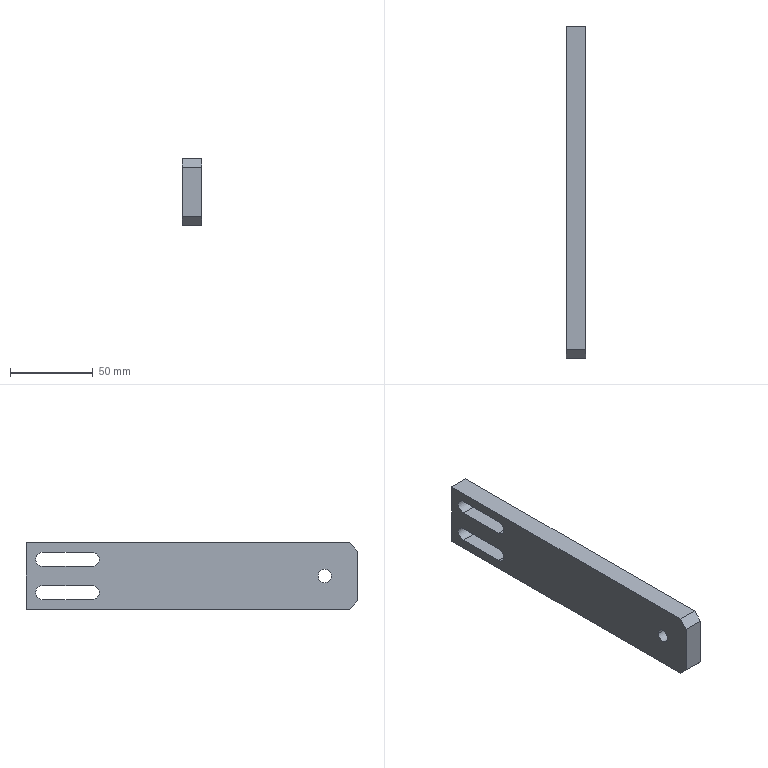Component | SolidWorks | ElectricalBoxAssembly2-1_GuidePlate2-1 | 1 solid | 20 faces | box 12 x 200 x 40 mm | volume 87615 mm3 | plane 12 | cylinder 8 | commonest cylinder face diameters 8.5 x6 8 x2
build123d program:
from build123d import *

# Parameters (mm, degrees)
SKETCH1_W           = 200
SKETCH1_H           = 40
BOSS_EXTRUDE1_DEPTH = 12
M8_TAPPED_HOLE1_D   = 8
CHAMFER1_SIZE       = 5
CHAMFER2_SIZE       = 5


with BuildPart() as part:
    # Sketch1 → Boss-Extrude1 (new body)
    with BuildSketch(Plane.XY):
        Rectangle(SKETCH1_W, SKETCH1_H)
        with BuildLine():
            Line((60, 14.25), (90, 14.25))
            ThreePointArc((90, 14.25), (94.25, 10), (90, 5.75))
            Line((90, 5.75), (60, 5.75))
            ThreePointArc((60, 5.75), (55.75, 10), (60, 14.25))
        make_face(mode=Mode.SUBTRACT)
        with BuildLine():
            Line((60, -5.75), (90, -5.75))
            ThreePointArc((90, -5.75), (94.25, -10), (90, -14.25))
            Line((90, -14.25), (60, -14.25))
            ThreePointArc((60, -14.25), (55.75, -10), (60, -5.75))
        make_face(mode=Mode.SUBTRACT)
    extrude(amount=BOSS_EXTRUDE1_DEPTH)

    # M8 Tapped Hole1 (through all)
    with Locations(Plane.XY.offset(12)):
        with Locations((-80, 0)):
            Hole(M8_TAPPED_HOLE1_D / 2)

    # Chamfer1
    chamfer1_edges = [part.edges().sort_by_distance(p)[0] for p in [
        (-100, 20, 6),
    ]]
    chamfer(chamfer1_edges, length=CHAMFER1_SIZE)

    # Chamfer2
    chamfer2_edges = [part.edges().sort_by_distance(p)[0] for p in [
        (-100, -20, 6),
    ]]
    chamfer(chamfer2_edges, length=CHAMFER2_SIZE)


solid = part.part

# Placed as in the assembly
solid = solid.moved(Location((743.468, 14.666, 1576.399), (90, 90, 0)))
STEP:
#1=CARTESIAN_POINT('',(29.743,-2.73,62.063));
#2=VERTEX_POINT('',#1);
#3=CARTESIAN_POINT('',(29.743,-2.415,62.063));
#4=VERTEX_POINT('',#3);
#5=CARTESIAN_POINT('',(29.743,-2.572,62.063));
#6=DIRECTION('',(-1.,-0.,-0.));
#7=DIRECTION('',(0.,1.,0.));
#8=AXIS2_PLACEMENT_3D('',#5,#6,#7);
#9=CIRCLE('',#8,0.1575);
#10=EDGE_CURVE('',#2,#4,#9,.T.);
#11=ORIENTED_EDGE('',*,*,#10,.F.);
#12=CARTESIAN_POINT('',(29.27,-2.73,62.063));
#13=VERTEX_POINT('',#12);
#14=CARTESIAN_POINT('',(29.27,-2.73,62.063));
#15=DIRECTION('',(-1.,-0.,-0.));
#16=VECTOR('',#15,39.37);
#17=LINE('',#14,#16);
#18=EDGE_CURVE('',#2,#13,#17,.T.);
#19=ORIENTED_EDGE('',*,*,#18,.T.);
#20=CARTESIAN_POINT('',(29.27,-2.415,62.063));
#21=VERTEX_POINT('',#20);
#22=CARTESIAN_POINT('',(29.27,-2.572,62.063));
#23=DIRECTION('',(-1.,-0.,-0.));
#24=DIRECTION('',(0.,1.,0.));
#25=AXIS2_PLACEMENT_3D('',#22,#23,#24);
#26=CIRCLE('',#25,0.1575);
#27=EDGE_CURVE('',#13,#21,#26,.T.);
#28=ORIENTED_EDGE('',*,*,#27,.T.);
#29=CARTESIAN_POINT('',(29.27,-2.415,62.063));
#30=DIRECTION('',(-1.,-0.,-0.));
#31=VECTOR('',#30,39.37);
#32=LINE('',#29,#31);
#33=EDGE_CURVE('',#4,#21,#32,.T.);
#34=ORIENTED_EDGE('',*,*,#33,.F.);
#35=EDGE_LOOP('',(#11,#19,#28,#34));
#36=FACE_OUTER_BOUND('',#35,.T.);
#37=CARTESIAN_POINT('',(29.27,-2.572,62.063));
#38=DIRECTION('',(-1.,-0.,-0.));
#39=DIRECTION('',(0.,1.,0.));
#40=AXIS2_PLACEMENT_3D('',#37,#38,#39);
#41=CYLINDRICAL_SURFACE('',#40,0.1575);
#42=ADVANCED_FACE('',(#36),#41,.F.);
#43=CARTESIAN_POINT('',(29.27,2.94,62.289));
#44=VERTEX_POINT('',#43);
#45=CARTESIAN_POINT('',(29.27,2.772,62.457));
#46=VERTEX_POINT('',#45);
#47=CARTESIAN_POINT('',(29.27,2.94,62.457));
#48=DIRECTION('',(-1.,-0.,-0.));
#49=DIRECTION('',(0.,1.,0.));
#50=AXIS2_PLACEMENT_3D('',#47,#48,#49);
#51=CIRCLE('',#50,0.1673);
#52=EDGE_CURVE('',#44,#46,#51,.T.);
#53=ORIENTED_EDGE('',*,*,#52,.T.);
#54=CARTESIAN_POINT('',(29.743,2.772,62.457));
#55=VERTEX_POINT('',#54);
#56=CARTESIAN_POINT('',(29.27,2.772,62.457));
#57=DIRECTION('',(1.,0.,0.));
#58=VECTOR('',#57,39.37);
#59=LINE('',#56,#58);
#60=EDGE_CURVE('',#46,#55,#59,.T.);
#61=ORIENTED_EDGE('',*,*,#60,.T.);
#62=CARTESIAN_POINT('',(29.743,2.94,62.289));
#63=VERTEX_POINT('',#62);
#64=CARTESIAN_POINT('',(29.743,2.94,62.457));
#65=DIRECTION('',(-1.,-0.,-0.));
#66=DIRECTION('',(0.,1.,0.));
#67=AXIS2_PLACEMENT_3D('',#64,#65,#66);
#68=CIRCLE('',#67,0.1673);
#69=EDGE_CURVE('',#63,#55,#68,.T.);
#70=ORIENTED_EDGE('',*,*,#69,.F.);
#71=CARTESIAN_POINT('',(29.27,2.94,62.289));
#72=DIRECTION('',(1.,0.,0.));
#73=VECTOR('',#72,39.37);
#74=LINE('',#71,#73);
#75=EDGE_CURVE('',#44,#63,#74,.T.);
#76=ORIENTED_EDGE('',*,*,#75,.F.);
#77=EDGE_LOOP('',(#53,#61,#70,#76));
#78=FACE_OUTER_BOUND('',#77,.T.);
#79=CARTESIAN_POINT('',(29.27,2.94,62.457));
#80=DIRECTION('',(1.,0.,0.));
#81=DIRECTION('',(0.,-1.,0.));
#82=AXIS2_PLACEMENT_3D('',#79,#80,#81);
#83=CYLINDRICAL_SURFACE('',#82,0.1673);
#84=ADVANCED_FACE('',(#78),#83,.F.);
#85=CARTESIAN_POINT('',(29.27,2.94,61.502));
#86=VERTEX_POINT('',#85);
#87=CARTESIAN_POINT('',(29.27,2.772,61.669));
#88=VERTEX_POINT('',#87);
#89=CARTESIAN_POINT('',(29.27,2.94,61.669));
#90=DIRECTION('',(-1.,-0.,-0.));
#91=DIRECTION('',(0.,1.,0.));
#92=AXIS2_PLACEMENT_3D('',#89,#90,#91);
#93=CIRCLE('',#92,0.1673);
#94=EDGE_CURVE('',#86,#88,#93,.T.);
#95=ORIENTED_EDGE('',*,*,#94,.T.);
#96=CARTESIAN_POINT('',(29.743,2.772,61.669));
#97=VERTEX_POINT('',#96);
#98=CARTESIAN_POINT('',(29.27,2.772,61.669));
#99=DIRECTION('',(1.,0.,0.));
#100=VECTOR('',#99,39.37);
#101=LINE('',#98,#100);
#102=EDGE_CURVE('',#88,#97,#101,.T.);
#103=ORIENTED_EDGE('',*,*,#102,.T.);
#104=CARTESIAN_POINT('',(29.743,2.94,61.502));
#105=VERTEX_POINT('',#104);
#106=CARTESIAN_POINT('',(29.743,2.94,61.669));
#107=DIRECTION('',(-1.,-0.,-0.));
#108=DIRECTION('',(0.,1.,0.));
#109=AXIS2_PLACEMENT_3D('',#106,#107,#108);
#110=CIRCLE('',#109,0.1673);
#111=EDGE_CURVE('',#105,#97,#110,.T.);
#112=ORIENTED_EDGE('',*,*,#111,.F.);
#113=CARTESIAN_POINT('',(29.27,2.94,61.502));
#114=DIRECTION('',(1.,0.,0.));
#115=VECTOR('',#114,39.37);
#116=LINE('',#113,#115);
#117=EDGE_CURVE('',#86,#105,#116,.T.);
#118=ORIENTED_EDGE('',*,*,#117,.F.);
#119=EDGE_LOOP('',(#95,#103,#112,#118));
#120=FACE_OUTER_BOUND('',#119,.T.);
#121=CARTESIAN_POINT('',(29.27,2.94,61.669));
#122=DIRECTION('',(1.,0.,0.));
#123=DIRECTION('',(0.,-1.,0.));
#124=AXIS2_PLACEMENT_3D('',#121,#122,#123);
#125=CYLINDRICAL_SURFACE('',#124,0.1673);
#126=ADVANCED_FACE('',(#120),#125,.F.);
#127=CARTESIAN_POINT('',(29.27,-2.572,62.063));
#128=DIRECTION('',(-1.,-0.,-0.));
#129=DIRECTION('',(0.,1.,0.));
#130=AXIS2_PLACEMENT_3D('',#127,#128,#129);
#131=CIRCLE('',#130,0.1575);
#132=EDGE_CURVE('',#21,#13,#131,.T.);
#133=ORIENTED_EDGE('',*,*,#132,.F.);
#134=ORIENTED_EDGE('',*,*,#27,.F.);
#135=EDGE_LOOP('',(#133,#134));
#136=FACE_BOUND('',#135,.T.);
#137=CARTESIAN_POINT('',(29.27,-3.36,61.472));
#138=VERTEX_POINT('',#137);
#139=CARTESIAN_POINT('',(29.27,-3.36,62.653));
#140=VERTEX_POINT('',#139);
#141=CARTESIAN_POINT('',(29.27,-3.36,61.276));
#142=DIRECTION('',(-0.,-0.,1.));
#143=VECTOR('',#142,39.37);
#144=LINE('',#141,#143);
#145=EDGE_CURVE('',#138,#140,#144,.T.);
#146=ORIENTED_EDGE('',*,*,#145,.T.);
#147=CARTESIAN_POINT('',(29.27,-3.163,62.85));
#148=VERTEX_POINT('',#147);
#149=CARTESIAN_POINT('',(29.27,-1.686,64.327));
#150=DIRECTION('',(-0.,0.7071,0.7071));
#151=VECTOR('',#150,39.37);
#152=LINE('',#149,#151);
#153=EDGE_CURVE('',#140,#148,#152,.T.);
#154=ORIENTED_EDGE('',*,*,#153,.T.);
#155=CARTESIAN_POINT('',(29.27,4.514,62.85));
#156=VERTEX_POINT('',#155);
#157=CARTESIAN_POINT('',(29.27,-3.36,62.85));
#158=DIRECTION('',(-0.,1.,0.));
#159=VECTOR('',#158,39.37);
#160=LINE('',#157,#159);
#161=EDGE_CURVE('',#148,#156,#160,.T.);
#162=ORIENTED_EDGE('',*,*,#161,.T.);
#163=CARTESIAN_POINT('',(29.27,4.514,61.276));
#164=VERTEX_POINT('',#163);
#165=CARTESIAN_POINT('',(29.27,4.514,61.276));
#166=DIRECTION('',(0.,0.,-1.));
#167=VECTOR('',#166,39.37);
#168=LINE('',#165,#167);
#169=EDGE_CURVE('',#156,#164,#168,.T.);
#170=ORIENTED_EDGE('',*,*,#169,.T.);
#171=CARTESIAN_POINT('',(29.27,-3.163,61.276));
#172=VERTEX_POINT('',#171);
#173=CARTESIAN_POINT('',(29.27,-3.36,61.276));
#174=DIRECTION('',(0.,-1.,-0.));
#175=VECTOR('',#174,39.37);
#176=LINE('',#173,#175);
#177=EDGE_CURVE('',#164,#172,#176,.T.);
#178=ORIENTED_EDGE('',*,*,#177,.T.);
#179=CARTESIAN_POINT('',(29.27,-1.686,59.799));
#180=DIRECTION('',(-0.,-0.7071,0.7071));
#181=VECTOR('',#180,39.37);
#182=LINE('',#179,#181);
#183=EDGE_CURVE('',#172,#138,#182,.T.);
#184=ORIENTED_EDGE('',*,*,#183,.T.);
#185=EDGE_LOOP('',(#146,#154,#162,#170,#178,#184));
#186=FACE_OUTER_BOUND('',#185,.T.);
#187=CARTESIAN_POINT('',(29.27,2.94,61.837));
#188=VERTEX_POINT('',#187);
#189=CARTESIAN_POINT('',(29.27,4.121,61.837));
#190=VERTEX_POINT('',#189);
#191=CARTESIAN_POINT('',(29.27,2.94,61.837));
#192=DIRECTION('',(-0.,1.,0.));
#193=VECTOR('',#192,39.37);
#194=LINE('',#191,#193);
#195=EDGE_CURVE('',#188,#190,#194,.T.);
#196=ORIENTED_EDGE('',*,*,#195,.F.);
#197=CARTESIAN_POINT('',(29.27,2.94,61.669));
#198=DIRECTION('',(-1.,-0.,-0.));
#199=DIRECTION('',(0.,1.,0.));
#200=AXIS2_PLACEMENT_3D('',#197,#198,#199);
#201=CIRCLE('',#200,0.1673);
#202=EDGE_CURVE('',#88,#188,#201,.T.);
#203=ORIENTED_EDGE('',*,*,#202,.F.);
#204=ORIENTED_EDGE('',*,*,#94,.F.);
#205=CARTESIAN_POINT('',(29.27,4.121,61.502));
#206=VERTEX_POINT('',#205);
#207=CARTESIAN_POINT('',(29.27,2.94,61.502));
#208=DIRECTION('',(0.,-1.,-0.));
#209=VECTOR('',#208,39.37);
#210=LINE('',#207,#209);
#211=EDGE_CURVE('',#206,#86,#210,.T.);
#212=ORIENTED_EDGE('',*,*,#211,.F.);
#213=CARTESIAN_POINT('',(29.27,4.121,61.669));
#214=DIRECTION('',(-1.,-0.,-0.));
#215=DIRECTION('',(0.,1.,0.));
#216=AXIS2_PLACEMENT_3D('',#213,#214,#215);
#217=CIRCLE('',#216,0.1673);
#218=EDGE_CURVE('',#190,#206,#217,.T.);
#219=ORIENTED_EDGE('',*,*,#218,.F.);
#220=EDGE_LOOP('',(#196,#203,#204,#212,#219));
#221=FACE_BOUND('',#220,.T.);
#222=CARTESIAN_POINT('',(29.27,2.94,62.624));
#223=VERTEX_POINT('',#222);
#224=CARTESIAN_POINT('',(29.27,4.121,62.624));
#225=VERTEX_POINT('',#224);
#226=CARTESIAN_POINT('',(29.27,2.94,62.624));
#227=DIRECTION('',(-0.,1.,0.));
#228=VECTOR('',#227,39.37);
#229=LINE('',#226,#228);
#230=EDGE_CURVE('',#223,#225,#229,.T.);
#231=ORIENTED_EDGE('',*,*,#230,.F.);
#232=CARTESIAN_POINT('',(29.27,2.94,62.457));
#233=DIRECTION('',(-1.,-0.,-0.));
#234=DIRECTION('',(0.,1.,0.));
#235=AXIS2_PLACEMENT_3D('',#232,#233,#234);
#236=CIRCLE('',#235,0.1673);
#237=EDGE_CURVE('',#46,#223,#236,.T.);
#238=ORIENTED_EDGE('',*,*,#237,.F.);
#239=ORIENTED_EDGE('',*,*,#52,.F.);
#240=CARTESIAN_POINT('',(29.27,4.121,62.289));
#241=VERTEX_POINT('',#240);
#242=CARTESIAN_POINT('',(29.27,2.94,62.289));
#243=DIRECTION('',(0.,-1.,-0.));
#244=VECTOR('',#243,39.37);
#245=LINE('',#242,#244);
#246=EDGE_CURVE('',#241,#44,#245,.T.);
#247=ORIENTED_EDGE('',*,*,#246,.F.);
#248=CARTESIAN_POINT('',(29.27,4.121,62.457));
#249=DIRECTION('',(-1.,-0.,-0.));
#250=DIRECTION('',(0.,1.,0.));
#251=AXIS2_PLACEMENT_3D('',#248,#249,#250);
#252=CIRCLE('',#251,0.1673);
#253=EDGE_CURVE('',#225,#241,#252,.T.);
#254=ORIENTED_EDGE('',*,*,#253,.F.);
#255=EDGE_LOOP('',(#231,#238,#239,#247,#254));
#256=FACE_BOUND('',#255,.T.);
#257=CARTESIAN_POINT('',(29.27,0.5774,62.063));
#258=DIRECTION('',(-1.,-0.,-0.));
#259=DIRECTION('',(-0.,1.,0.));
#260=AXIS2_PLACEMENT_3D('',#257,#258,#259);
#261=PLANE('',#260);
#262=ADVANCED_FACE('',(#136,#186,#221,#256),#261,.T.);
#263=CARTESIAN_POINT('',(29.743,-2.572,62.063));
#264=DIRECTION('',(-1.,-0.,-0.));
#265=DIRECTION('',(0.,1.,0.));
#266=AXIS2_PLACEMENT_3D('',#263,#264,#265);
#267=CIRCLE('',#266,0.1575);
#268=EDGE_CURVE('',#4,#2,#267,.T.);
#269=ORIENTED_EDGE('',*,*,#268,.T.);
#270=ORIENTED_EDGE('',*,*,#10,.T.);
#271=EDGE_LOOP('',(#269,#270));
#272=FACE_BOUND('',#271,.T.);
#273=ORIENTED_EDGE('',*,*,#111,.T.);
#274=CARTESIAN_POINT('',(29.743,2.94,61.837));
#275=VERTEX_POINT('',#274);
#276=CARTESIAN_POINT('',(29.743,2.94,61.669));
#277=DIRECTION('',(-1.,-0.,-0.));
#278=DIRECTION('',(0.,1.,0.));
#279=AXIS2_PLACEMENT_3D('',#276,#277,#278);
#280=CIRCLE('',#279,0.1673);
#281=EDGE_CURVE('',#97,#275,#280,.T.);
#282=ORIENTED_EDGE('',*,*,#281,.T.);
#283=CARTESIAN_POINT('',(29.743,4.121,61.837));
#284=VERTEX_POINT('',#283);
#285=CARTESIAN_POINT('',(29.743,2.94,61.837));
#286=DIRECTION('',(-0.,1.,0.));
#287=VECTOR('',#286,39.37);
#288=LINE('',#285,#287);
#289=EDGE_CURVE('',#275,#284,#288,.T.);
#290=ORIENTED_EDGE('',*,*,#289,.T.);
#291=CARTESIAN_POINT('',(29.743,4.121,61.502));
#292=VERTEX_POINT('',#291);
#293=CARTESIAN_POINT('',(29.743,4.121,61.669));
#294=DIRECTION('',(-1.,-0.,-0.));
#295=DIRECTION('',(0.,1.,0.));
#296=AXIS2_PLACEMENT_3D('',#293,#294,#295);
#297=CIRCLE('',#296,0.1673);
#298=EDGE_CURVE('',#284,#292,#297,.T.);
#299=ORIENTED_EDGE('',*,*,#298,.T.);
#300=CARTESIAN_POINT('',(29.743,2.94,61.502));
#301=DIRECTION('',(0.,-1.,-0.));
#302=VECTOR('',#301,39.37);
#303=LINE('',#300,#302);
#304=EDGE_CURVE('',#292,#105,#303,.T.);
#305=ORIENTED_EDGE('',*,*,#304,.T.);
#306=EDGE_LOOP('',(#273,#282,#290,#299,#305));
#307=FACE_BOUND('',#306,.T.);
#308=CARTESIAN_POINT('',(29.743,-3.163,62.85));
#309=VERTEX_POINT('',#308);
#310=CARTESIAN_POINT('',(29.743,4.514,62.85));
#311=VERTEX_POINT('',#310);
#312=CARTESIAN_POINT('',(29.743,-3.36,62.85));
#313=DIRECTION('',(-0.,1.,0.));
#314=VECTOR('',#313,39.37);
#315=LINE('',#312,#314);
#316=EDGE_CURVE('',#309,#311,#315,.T.);
#317=ORIENTED_EDGE('',*,*,#316,.F.);
#318=CARTESIAN_POINT('',(29.743,-3.36,62.653));
#319=VERTEX_POINT('',#318);
#320=CARTESIAN_POINT('',(29.743,-3.163,62.85));
#321=DIRECTION('',(0.,-0.7071,-0.7071));
#322=VECTOR('',#321,39.37);
#323=LINE('',#320,#322);
#324=EDGE_CURVE('',#309,#319,#323,.T.);
#325=ORIENTED_EDGE('',*,*,#324,.T.);
#326=CARTESIAN_POINT('',(29.743,-3.36,61.472));
#327=VERTEX_POINT('',#326);
#328=CARTESIAN_POINT('',(29.743,-3.36,61.276));
#329=DIRECTION('',(-0.,-0.,1.));
#330=VECTOR('',#329,39.37);
#331=LINE('',#328,#330);
#332=EDGE_CURVE('',#327,#319,#331,.T.);
#333=ORIENTED_EDGE('',*,*,#332,.F.);
#334=CARTESIAN_POINT('',(29.743,-3.163,61.276));
#335=VERTEX_POINT('',#334);
#336=CARTESIAN_POINT('',(29.743,-3.36,61.472));
#337=DIRECTION('',(0.,0.7071,-0.7071));
#338=VECTOR('',#337,39.37);
#339=LINE('',#336,#338);
#340=EDGE_CURVE('',#327,#335,#339,.T.);
#341=ORIENTED_EDGE('',*,*,#340,.T.);
#342=CARTESIAN_POINT('',(29.743,4.514,61.276));
#343=VERTEX_POINT('',#342);
#344=CARTESIAN_POINT('',(29.743,-3.36,61.276));
#345=DIRECTION('',(0.,-1.,-0.));
#346=VECTOR('',#345,39.37);
#347=LINE('',#344,#346);
#348=EDGE_CURVE('',#343,#335,#347,.T.);
#349=ORIENTED_EDGE('',*,*,#348,.F.);
#350=CARTESIAN_POINT('',(29.743,4.514,61.276));
#351=DIRECTION('',(0.,0.,-1.));
#352=VECTOR('',#351,39.37);
#353=LINE('',#350,#352);
#354=EDGE_CURVE('',#311,#343,#353,.T.);
#355=ORIENTED_EDGE('',*,*,#354,.F.);
#356=EDGE_LOOP('',(#317,#325,#333,#341,#349,#355));
#357=FACE_OUTER_BOUND('',#356,.T.);
#358=ORIENTED_EDGE('',*,*,#69,.T.);
#359=CARTESIAN_POINT('',(29.743,2.94,62.624));
#360=VERTEX_POINT('',#359);
#361=CARTESIAN_POINT('',(29.743,2.94,62.457));
#362=DIRECTION('',(-1.,-0.,-0.));
#363=DIRECTION('',(0.,1.,0.));
#364=AXIS2_PLACEMENT_3D('',#361,#362,#363);
#365=CIRCLE('',#364,0.1673);
#366=EDGE_CURVE('',#55,#360,#365,.T.);
#367=ORIENTED_EDGE('',*,*,#366,.T.);
#368=CARTESIAN_POINT('',(29.743,4.121,62.624));
#369=VERTEX_POINT('',#368);
#370=CARTESIAN_POINT('',(29.743,2.94,62.624));
#371=DIRECTION('',(-0.,1.,0.));
#372=VECTOR('',#371,39.37);
#373=LINE('',#370,#372);
#374=EDGE_CURVE('',#360,#369,#373,.T.);
#375=ORIENTED_EDGE('',*,*,#374,.T.);
#376=CARTESIAN_POINT('',(29.743,4.121,62.289));
#377=VERTEX_POINT('',#376);
#378=CARTESIAN_POINT('',(29.743,4.121,62.457));
#379=DIRECTION('',(-1.,-0.,-0.));
#380=DIRECTION('',(0.,1.,0.));
#381=AXIS2_PLACEMENT_3D('',#378,#379,#380);
#382=CIRCLE('',#381,0.1673);
#383=EDGE_CURVE('',#369,#377,#382,.T.);
#384=ORIENTED_EDGE('',*,*,#383,.T.);
#385=CARTESIAN_POINT('',(29.743,2.94,62.289));
#386=DIRECTION('',(0.,-1.,-0.));
#387=VECTOR('',#386,39.37);
#388=LINE('',#385,#387);
#389=EDGE_CURVE('',#377,#63,#388,.T.);
#390=ORIENTED_EDGE('',*,*,#389,.T.);
#391=EDGE_LOOP('',(#358,#367,#375,#384,#390));
#392=FACE_BOUND('',#391,.T.);
#393=CARTESIAN_POINT('',(29.743,0.5774,62.063));
#394=DIRECTION('',(-1.,-0.,-0.));
#395=DIRECTION('',(-0.,1.,0.));
#396=AXIS2_PLACEMENT_3D('',#393,#394,#395);
#397=PLANE('',#396);
#398=ADVANCED_FACE('',(#272,#307,#357,#392),#397,.F.);
#399=ORIENTED_EDGE('',*,*,#354,.T.);
#400=CARTESIAN_POINT('',(29.27,4.514,61.276));
#401=DIRECTION('',(1.,0.,0.));
#402=VECTOR('',#401,39.37);
#403=LINE('',#400,#402);
#404=EDGE_CURVE('',#164,#343,#403,.T.);
#405=ORIENTED_EDGE('',*,*,#404,.F.);
#406=ORIENTED_EDGE('',*,*,#169,.F.);
#407=CARTESIAN_POINT('',(29.27,4.514,62.85));
#408=DIRECTION('',(1.,0.,0.));
#409=VECTOR('',#408,39.37);
#410=LINE('',#407,#409);
#411=EDGE_CURVE('',#156,#311,#410,.T.);
#412=ORIENTED_EDGE('',*,*,#411,.T.);
#413=EDGE_LOOP('',(#399,#405,#406,#412));
#414=FACE_OUTER_BOUND('',#413,.T.);
#415=CARTESIAN_POINT('',(29.27,4.514,61.276));
#416=DIRECTION('',(0.,-1.,-0.));
#417=DIRECTION('',(-1.,-0.,-0.));
#418=AXIS2_PLACEMENT_3D('',#415,#416,#417);
#419=PLANE('',#418);
#420=ADVANCED_FACE('',(#414),#419,.F.);
#421=ORIENTED_EDGE('',*,*,#348,.T.);
#422=CARTESIAN_POINT('',(29.27,-3.163,61.276));
#423=DIRECTION('',(-1.,-0.,-0.));
#424=VECTOR('',#423,39.37);
#425=LINE('',#422,#424);
#426=EDGE_CURVE('',#335,#172,#425,.T.);
#427=ORIENTED_EDGE('',*,*,#426,.T.);
#428=ORIENTED_EDGE('',*,*,#177,.F.);
#429=ORIENTED_EDGE('',*,*,#404,.T.);
#430=EDGE_LOOP('',(#421,#427,#428,#429));
#431=FACE_OUTER_BOUND('',#430,.T.);
#432=CARTESIAN_POINT('',(29.27,-3.36,61.276));
#433=DIRECTION('',(-0.,-0.,1.));
#434=DIRECTION('',(1.,0.,0.));
#435=AXIS2_PLACEMENT_3D('',#432,#433,#434);
#436=PLANE('',#435);
#437=ADVANCED_FACE('',(#431),#436,.F.);
#438=ORIENTED_EDGE('',*,*,#332,.T.);
#439=CARTESIAN_POINT('',(29.27,-3.36,62.653));
#440=DIRECTION('',(-1.,-0.,-0.));
#441=VECTOR('',#440,39.37);
#442=LINE('',#439,#441);
#443=EDGE_CURVE('',#319,#140,#442,.T.);
#444=ORIENTED_EDGE('',*,*,#443,.T.);
#445=ORIENTED_EDGE('',*,*,#145,.F.);
#446=CARTESIAN_POINT('',(29.27,-3.36,61.472));
#447=DIRECTION('',(1.,0.,0.));
#448=VECTOR('',#447,39.37);
#449=LINE('',#446,#448);
#450=EDGE_CURVE('',#138,#327,#449,.T.);
#451=ORIENTED_EDGE('',*,*,#450,.T.);
#452=EDGE_LOOP('',(#438,#444,#445,#451));
#453=FACE_OUTER_BOUND('',#452,.T.);
#454=CARTESIAN_POINT('',(29.27,-3.36,61.276));
#455=DIRECTION('',(-0.,1.,0.));
#456=DIRECTION('',(1.,0.,0.));
#457=AXIS2_PLACEMENT_3D('',#454,#455,#456);
#458=PLANE('',#457);
#459=ADVANCED_FACE('',(#453),#458,.F.);
#460=ORIENTED_EDGE('',*,*,#161,.F.);
#461=CARTESIAN_POINT('',(29.27,-3.163,62.85));
#462=DIRECTION('',(1.,0.,0.));
#463=VECTOR('',#462,39.37);
#464=LINE('',#461,#463);
#465=EDGE_CURVE('',#148,#309,#464,.T.);
#466=ORIENTED_EDGE('',*,*,#465,.T.);
#467=ORIENTED_EDGE('',*,*,#316,.T.);
#468=ORIENTED_EDGE('',*,*,#411,.F.);
#469=EDGE_LOOP('',(#460,#466,#467,#468));
#470=FACE_OUTER_BOUND('',#469,.T.);
#471=CARTESIAN_POINT('',(29.27,-3.36,62.85));
#472=DIRECTION('',(0.,0.,-1.));
#473=DIRECTION('',(-1.,-0.,-0.));
#474=AXIS2_PLACEMENT_3D('',#471,#472,#473);
#475=PLANE('',#474);
#476=ADVANCED_FACE('',(#470),#475,.F.);
#477=ORIENTED_EDGE('',*,*,#102,.F.);
#478=ORIENTED_EDGE('',*,*,#202,.T.);
#479=CARTESIAN_POINT('',(29.27,2.94,61.837));
#480=DIRECTION('',(1.,0.,0.));
#481=VECTOR('',#480,39.37);
#482=LINE('',#479,#481);
#483=EDGE_CURVE('',#188,#275,#482,.T.);
#484=ORIENTED_EDGE('',*,*,#483,.T.);
#485=ORIENTED_EDGE('',*,*,#281,.F.);
#486=EDGE_LOOP('',(#477,#478,#484,#485));
#487=FACE_OUTER_BOUND('',#486,.T.);
#488=CARTESIAN_POINT('',(29.27,2.94,61.669));
#489=DIRECTION('',(1.,0.,0.));
#490=DIRECTION('',(0.,-1.,0.));
#491=AXIS2_PLACEMENT_3D('',#488,#489,#490);
#492=CYLINDRICAL_SURFACE('',#491,0.1673);
#493=ADVANCED_FACE('',(#487),#492,.F.);
#494=ORIENTED_EDGE('',*,*,#289,.F.);
#495=ORIENTED_EDGE('',*,*,#483,.F.);
#496=ORIENTED_EDGE('',*,*,#195,.T.);
#497=CARTESIAN_POINT('',(29.27,4.121,61.837));
#498=DIRECTION('',(1.,0.,0.));
#499=VECTOR('',#498,39.37);
#500=LINE('',#497,#499);
#501=EDGE_CURVE('',#190,#284,#500,.T.);
#502=ORIENTED_EDGE('',*,*,#501,.T.);
#503=EDGE_LOOP('',(#494,#495,#496,#502));
#504=FACE_OUTER_BOUND('',#503,.T.);
#505=CARTESIAN_POINT('',(29.27,2.94,61.837));
#506=DIRECTION('',(0.,0.,-1.));
#507=DIRECTION('',(-1.,-0.,-0.));
#508=AXIS2_PLACEMENT_3D('',#505,#506,#507);
#509=PLANE('',#508);
#510=ADVANCED_FACE('',(#504),#509,.T.);
#511=ORIENTED_EDGE('',*,*,#298,.F.);
#512=ORIENTED_EDGE('',*,*,#501,.F.);
#513=ORIENTED_EDGE('',*,*,#218,.T.);
#514=CARTESIAN_POINT('',(29.27,4.121,61.502));
#515=DIRECTION('',(1.,0.,0.));
#516=VECTOR('',#515,39.37);
#517=LINE('',#514,#516);
#518=EDGE_CURVE('',#206,#292,#517,.T.);
#519=ORIENTED_EDGE('',*,*,#518,.T.);
#520=EDGE_LOOP('',(#511,#512,#513,#519));
#521=FACE_OUTER_BOUND('',#520,.T.);
#522=CARTESIAN_POINT('',(29.27,4.121,61.669));
#523=DIRECTION('',(1.,0.,0.));
#524=DIRECTION('',(0.,-1.,0.));
#525=AXIS2_PLACEMENT_3D('',#522,#523,#524);
#526=CYLINDRICAL_SURFACE('',#525,0.1673);
#527=ADVANCED_FACE('',(#521),#526,.F.);
#528=ORIENTED_EDGE('',*,*,#304,.F.);
#529=ORIENTED_EDGE('',*,*,#518,.F.);
#530=ORIENTED_EDGE('',*,*,#211,.T.);
#531=ORIENTED_EDGE('',*,*,#117,.T.);
#532=EDGE_LOOP('',(#528,#529,#530,#531));
#533=FACE_OUTER_BOUND('',#532,.T.);
#534=CARTESIAN_POINT('',(29.27,2.94,61.502));
#535=DIRECTION('',(-0.,-0.,1.));
#536=DIRECTION('',(1.,0.,0.));
#537=AXIS2_PLACEMENT_3D('',#534,#535,#536);
#538=PLANE('',#537);
#539=ADVANCED_FACE('',(#533),#538,.T.);
#540=ORIENTED_EDGE('',*,*,#60,.F.);
#541=ORIENTED_EDGE('',*,*,#237,.T.);
#542=CARTESIAN_POINT('',(29.27,2.94,62.624));
#543=DIRECTION('',(1.,0.,0.));
#544=VECTOR('',#543,39.37);
#545=LINE('',#542,#544);
#546=EDGE_CURVE('',#223,#360,#545,.T.);
#547=ORIENTED_EDGE('',*,*,#546,.T.);
#548=ORIENTED_EDGE('',*,*,#366,.F.);
#549=EDGE_LOOP('',(#540,#541,#547,#548));
#550=FACE_OUTER_BOUND('',#549,.T.);
#551=CARTESIAN_POINT('',(29.27,2.94,62.457));
#552=DIRECTION('',(1.,0.,0.));
#553=DIRECTION('',(0.,-1.,0.));
#554=AXIS2_PLACEMENT_3D('',#551,#552,#553);
#555=CYLINDRICAL_SURFACE('',#554,0.1673);
#556=ADVANCED_FACE('',(#550),#555,.F.);
#557=ORIENTED_EDGE('',*,*,#374,.F.);
#558=ORIENTED_EDGE('',*,*,#546,.F.);
#559=ORIENTED_EDGE('',*,*,#230,.T.);
#560=CARTESIAN_POINT('',(29.27,4.121,62.624));
#561=DIRECTION('',(1.,0.,0.));
#562=VECTOR('',#561,39.37);
#563=LINE('',#560,#562);
#564=EDGE_CURVE('',#225,#369,#563,.T.);
#565=ORIENTED_EDGE('',*,*,#564,.T.);
#566=EDGE_LOOP('',(#557,#558,#559,#565));
#567=FACE_OUTER_BOUND('',#566,.T.);
#568=CARTESIAN_POINT('',(29.27,2.94,62.624));
#569=DIRECTION('',(0.,0.,-1.));
#570=DIRECTION('',(-1.,-0.,-0.));
#571=AXIS2_PLACEMENT_3D('',#568,#569,#570);
#572=PLANE('',#571);
#573=ADVANCED_FACE('',(#567),#572,.T.);
#574=ORIENTED_EDGE('',*,*,#383,.F.);
#575=ORIENTED_EDGE('',*,*,#564,.F.);
#576=ORIENTED_EDGE('',*,*,#253,.T.);
#577=CARTESIAN_POINT('',(29.27,4.121,62.289));
#578=DIRECTION('',(1.,0.,0.));
#579=VECTOR('',#578,39.37);
#580=LINE('',#577,#579);
#581=EDGE_CURVE('',#241,#377,#580,.T.);
#582=ORIENTED_EDGE('',*,*,#581,.T.);
#583=EDGE_LOOP('',(#574,#575,#576,#582));
#584=FACE_OUTER_BOUND('',#583,.T.);
#585=CARTESIAN_POINT('',(29.27,4.121,62.457));
#586=DIRECTION('',(1.,0.,0.));
#587=DIRECTION('',(0.,-1.,0.));
#588=AXIS2_PLACEMENT_3D('',#585,#586,#587);
#589=CYLINDRICAL_SURFACE('',#588,0.1673);
#590=ADVANCED_FACE('',(#584),#589,.F.);
#591=ORIENTED_EDGE('',*,*,#389,.F.);
#592=ORIENTED_EDGE('',*,*,#581,.F.);
#593=ORIENTED_EDGE('',*,*,#246,.T.);
#594=ORIENTED_EDGE('',*,*,#75,.T.);
#595=EDGE_LOOP('',(#591,#592,#593,#594));
#596=FACE_OUTER_BOUND('',#595,.T.);
#597=CARTESIAN_POINT('',(29.27,2.94,62.289));
#598=DIRECTION('',(-0.,-0.,1.));
#599=DIRECTION('',(1.,0.,0.));
#600=AXIS2_PLACEMENT_3D('',#597,#598,#599);
#601=PLANE('',#600);
#602=ADVANCED_FACE('',(#596),#601,.T.);
#603=ORIENTED_EDGE('',*,*,#18,.F.);
#604=ORIENTED_EDGE('',*,*,#268,.F.);
#605=ORIENTED_EDGE('',*,*,#33,.T.);
#606=ORIENTED_EDGE('',*,*,#132,.T.);
#607=EDGE_LOOP('',(#603,#604,#605,#606));
#608=FACE_OUTER_BOUND('',#607,.T.);
#609=CARTESIAN_POINT('',(29.27,-2.572,62.063));
#610=DIRECTION('',(-1.,-0.,-0.));
#611=DIRECTION('',(0.,1.,0.));
#612=AXIS2_PLACEMENT_3D('',#609,#610,#611);
#613=CYLINDRICAL_SURFACE('',#612,0.1575);
#614=ADVANCED_FACE('',(#608),#613,.F.);
#615=ORIENTED_EDGE('',*,*,#183,.F.);
#616=ORIENTED_EDGE('',*,*,#426,.F.);
#617=ORIENTED_EDGE('',*,*,#340,.F.);
#618=ORIENTED_EDGE('',*,*,#450,.F.);
#619=EDGE_LOOP('',(#615,#616,#617,#618));
#620=FACE_OUTER_BOUND('',#619,.T.);
#621=CARTESIAN_POINT('',(29.27,-3.36,61.472));
#622=DIRECTION('',(-0.,0.7071,0.7071));
#623=DIRECTION('',(1.,0.,0.));
#624=AXIS2_PLACEMENT_3D('',#621,#622,#623);
#625=PLANE('',#624);
#626=ADVANCED_FACE('',(#620),#625,.F.);
#627=ORIENTED_EDGE('',*,*,#153,.F.);
#628=ORIENTED_EDGE('',*,*,#443,.F.);
#629=ORIENTED_EDGE('',*,*,#324,.F.);
#630=ORIENTED_EDGE('',*,*,#465,.F.);
#631=EDGE_LOOP('',(#627,#628,#629,#630));
#632=FACE_OUTER_BOUND('',#631,.T.);
#633=CARTESIAN_POINT('',(29.27,-3.163,62.85));
#634=DIRECTION('',(0.,0.7071,-0.7071));
#635=DIRECTION('',(1.,0.,0.));
#636=AXIS2_PLACEMENT_3D('',#633,#634,#635);
#637=PLANE('',#636);
#638=ADVANCED_FACE('',(#632),#637,.F.);
#639=CLOSED_SHELL('',(#42,#84,#126,#262,#398,#420,#437,#459,#476,#493,#510,#527,#539,#556,#573,#590,#602,#614,#626,#638));
#640=MANIFOLD_SOLID_BREP('',#639);
#641=CARTESIAN_POINT('',(0.,0.,0.));
#642=DIRECTION('',(0.,0.,1.));
#643=DIRECTION('',(1.,0.,0.));
#644=AXIS2_PLACEMENT_3D('',#641,#642,#643);
#645=(LENGTH_UNIT()NAMED_UNIT(*)SI_UNIT($,.METRE.));
#646=LENGTH_MEASURE_WITH_UNIT(LENGTH_MEASURE(0.0254),#645);
#647=DIMENSIONAL_EXPONENTS(1.,0.,0.,0.,0.,0.,0.);
#648=(CONVERSION_BASED_UNIT('',#646)LENGTH_UNIT()NAMED_UNIT(#647));
#649=UNCERTAINTY_MEASURE_WITH_UNIT(LENGTH_MEASURE(0.00001),#648,'','');
#650=(NAMED_UNIT(*)PLANE_ANGLE_UNIT()SI_UNIT($,.RADIAN.));
#651=(NAMED_UNIT(*)SI_UNIT($,.STERADIAN.)SOLID_ANGLE_UNIT());
#652=(GEOMETRIC_REPRESENTATION_CONTEXT(3)GLOBAL_UNCERTAINTY_ASSIGNED_CONTEXT((#649))GLOBAL_UNIT_ASSIGNED_CONTEXT((#648,#650,#651))REPRESENTATION_CONTEXT('',''));
#653=ADVANCED_BREP_SHAPE_REPRESENTATION('',(#640,#644),#652);
#654=COLOUR_RGB('',0.7922,0.8196,0.9333);
#655=FILL_AREA_STYLE_COLOUR('',#654);
#656=FILL_AREA_STYLE('',(#655));
#657=SURFACE_STYLE_FILL_AREA(#656);
#658=SURFACE_SIDE_STYLE('',(#657));
#659=SURFACE_STYLE_USAGE(.BOTH.,#658);
#660=PRESENTATION_STYLE_ASSIGNMENT((#659));
#661=STYLED_ITEM('',(#660),#640);
#662=(LENGTH_UNIT()NAMED_UNIT(*)SI_UNIT($,.METRE.));
#663=LENGTH_MEASURE_WITH_UNIT(LENGTH_MEASURE(0.0254),#662);
#664=DIMENSIONAL_EXPONENTS(1.,0.,0.,0.,0.,0.,0.);
#665=(CONVERSION_BASED_UNIT('',#663)LENGTH_UNIT()NAMED_UNIT(#664));
#666=UNCERTAINTY_MEASURE_WITH_UNIT(LENGTH_MEASURE(0.00001),#665,'','');
#667=(NAMED_UNIT(*)PLANE_ANGLE_UNIT()SI_UNIT($,.RADIAN.));
#668=(NAMED_UNIT(*)SI_UNIT($,.STERADIAN.)SOLID_ANGLE_UNIT());
#669=(GEOMETRIC_REPRESENTATION_CONTEXT(3)GLOBAL_UNCERTAINTY_ASSIGNED_CONTEXT((#666))GLOBAL_UNIT_ASSIGNED_CONTEXT((#665,#667,#668))REPRESENTATION_CONTEXT('',''));
#670=MECHANICAL_DESIGN_GEOMETRIC_PRESENTATION_REPRESENTATION('',(#661),#669);
#671=PRESENTATION_LAYER_ASSIGNMENT('','',(#661));